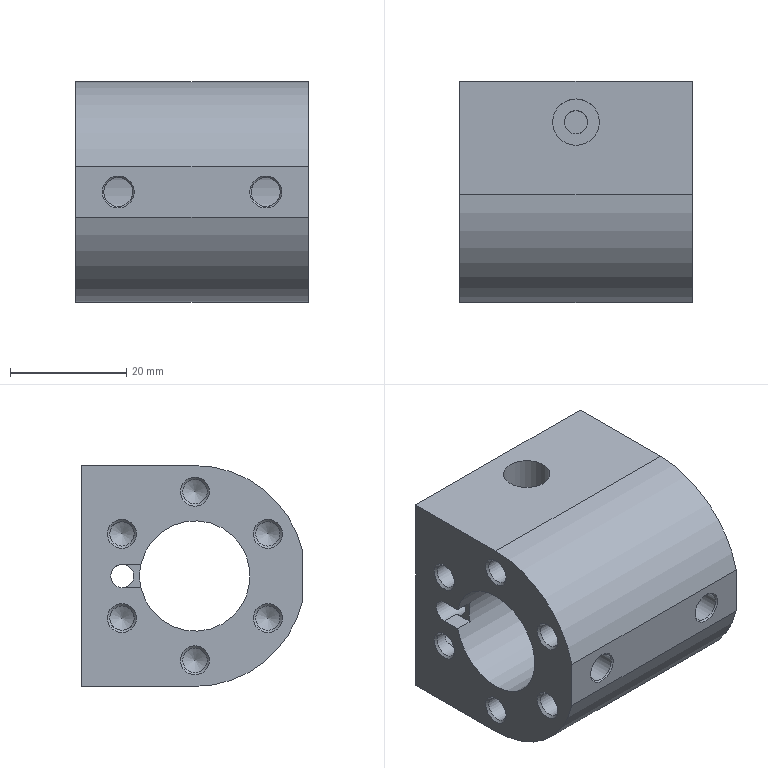Component | NX | PISTON_CYLINDER | 1 solid | 103 faces | volume 36020 mm3 | cone 42 | cylinder 38 | plane 23 | commonest cylinder face diameters 4.2 x12 3.3 x8 4 x6 5 x4 2.5 x4 38 x2 19 x1 8 x1